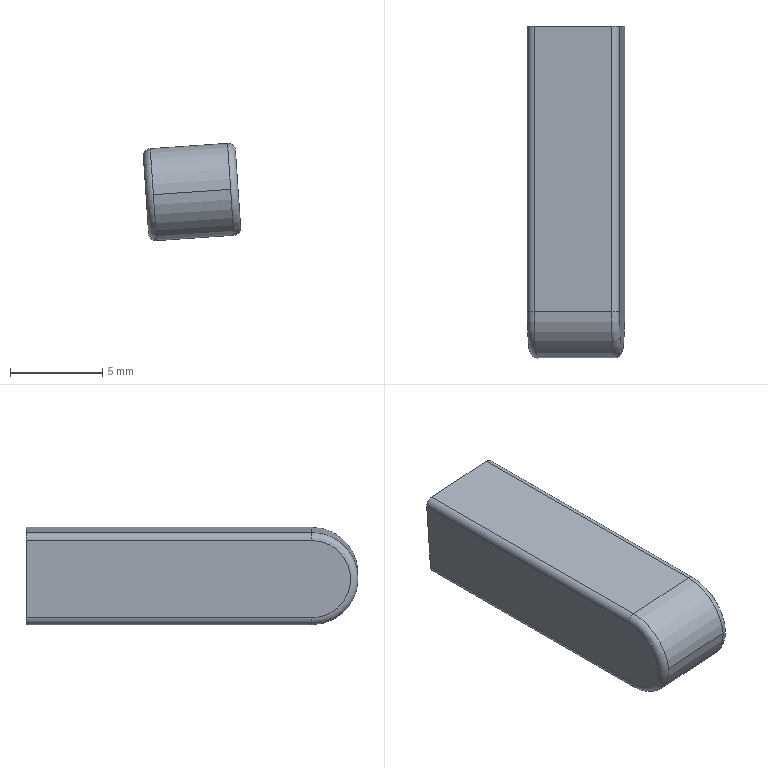Component | SolidWorks | GB_T1096-1979PlainParallelKeyC-type5_18-2 | 1 solid | 13 faces | box 5.28 x 18 x 5.28 mm | volume 434 mm3 | cylinder 6 | plane 5 | torus 2 | commonest cylinder face diameters 0.8 x4 5 x2
build123d program:
from build123d import *

# Parameters (mm, degrees)
BASE_EXTRUDE_DEPTH = 5
FILLET1_R          = 0.4


with BuildPart() as part:
    # Sketch1 → Base-Extrude (new body)
    with BuildSketch(Plane.XY):
        with BuildLine():
            Line((-9, 2.5), (6.5, 2.5))
            Line((6.5, 2.5), (6.5, -2.5))
            Line((6.5, -2.5), (-9, -2.5))
            ThreePointArc((-9, -2.5), (-11.5, 0), (-9, 2.5))
        make_face()
    extrude(amount=BASE_EXTRUDE_DEPTH)

    # Fillet1
    fillet1_edges = [part.edges().sort_by_distance(p)[0] for p in [
        (-11.5, 0, 5),
        (-1.25, -2.5, 5),
        (-1.25, -2.5, 0),
        (-11.5, 0, 0),
        (-1.25, 2.5, 0),
        (-1.25, 2.5, 5),
    ]]
    fillet(fillet1_edges, radius=FILLET1_R)


solid = part.part

# Placed as in the assembly
solid = solid.moved(Location((-24.351, 150.766, -166.303), (0, 86.093, 90)))
STEP:
#1=CARTESIAN_POINT('',(-0.7713,5.581,-6.633));
#2=VERTEX_POINT('',#1);
#3=CARTESIAN_POINT('',(-0.778,5.483,-6.535));
#4=VERTEX_POINT('',#3);
#5=CARTESIAN_POINT('',(-0.778,5.581,-6.535));
#6=DIRECTION('',(-0.9977,-0.,-0.06814));
#7=DIRECTION('',(0.,1.,0.));
#8=AXIS2_PLACEMENT_3D('',#5,#6,#7);
#9=CIRCLE('',#8,0.09843);
#10=EDGE_CURVE('',#2,#4,#9,.T.);
#11=ORIENTED_EDGE('',*,*,#10,.T.);
#12=CARTESIAN_POINT('',(-0.943,5.483,-6.546));
#13=VERTEX_POINT('',#12);
#14=CARTESIAN_POINT('',(-0.7623,5.483,-6.534));
#15=DIRECTION('',(-0.9977,-0.,-0.06814));
#16=VECTOR('',#15,39.37);
#17=LINE('',#14,#16);
#18=EDGE_CURVE('',#4,#13,#17,.T.);
#19=ORIENTED_EDGE('',*,*,#18,.T.);
#20=CARTESIAN_POINT('',(-0.9363,5.581,-6.644));
#21=VERTEX_POINT('',#20);
#22=CARTESIAN_POINT('',(-0.943,5.581,-6.546));
#23=DIRECTION('',(0.9977,0.,0.06814));
#24=DIRECTION('',(0.,1.,0.));
#25=AXIS2_PLACEMENT_3D('',#22,#23,#24);
#26=CIRCLE('',#25,0.09843);
#27=EDGE_CURVE('',#13,#21,#26,.T.);
#28=ORIENTED_EDGE('',*,*,#27,.T.);
#29=CARTESIAN_POINT('',(-0.7556,5.581,-6.632));
#30=DIRECTION('',(-0.9977,-0.,-0.06814));
#31=VECTOR('',#30,39.37);
#32=LINE('',#29,#31);
#33=EDGE_CURVE('',#2,#21,#32,.T.);
#34=ORIENTED_EDGE('',*,*,#33,.F.);
#35=EDGE_LOOP('',(#11,#19,#28,#34));
#36=FACE_OUTER_BOUND('',#35,.T.);
#37=CARTESIAN_POINT('',(-0.7623,5.581,-6.534));
#38=DIRECTION('',(-0.9977,-0.,-0.06814));
#39=DIRECTION('',(0.,-1.,0.));
#40=AXIS2_PLACEMENT_3D('',#37,#38,#39);
#41=CYLINDRICAL_SURFACE('',#40,0.09843);
#42=ADVANCED_FACE('',(#36),#41,.T.);
#43=CARTESIAN_POINT('',(-0.7567,6.192,-6.616));
#44=VERTEX_POINT('',#43);
#45=CARTESIAN_POINT('',(-0.768,6.192,-6.451));
#46=VERTEX_POINT('',#45);
#47=CARTESIAN_POINT('',(-0.769,6.192,-6.436));
#48=DIRECTION('',(-0.06814,0.,0.9977));
#49=VECTOR('',#48,39.37);
#50=LINE('',#47,#49);
#51=EDGE_CURVE('',#44,#46,#50,.T.);
#52=ORIENTED_EDGE('',*,*,#51,.F.);
#53=CARTESIAN_POINT('',(-0.7713,6.192,-6.633));
#54=VERTEX_POINT('',#53);
#55=CARTESIAN_POINT('',(-0.7724,6.192,-6.617));
#56=DIRECTION('',(0.,1.,-0.));
#57=DIRECTION('',(0.9977,0.,0.06814));
#58=AXIS2_PLACEMENT_3D('',#55,#56,#57);
#59=CIRCLE('',#58,0.01575);
#60=EDGE_CURVE('',#44,#54,#59,.T.);
#61=ORIENTED_EDGE('',*,*,#60,.T.);
#62=CARTESIAN_POINT('',(-0.9363,6.192,-6.644));
#63=VERTEX_POINT('',#62);
#64=CARTESIAN_POINT('',(-0.7556,6.192,-6.632));
#65=DIRECTION('',(-0.9977,-0.,-0.06814));
#66=VECTOR('',#65,39.37);
#67=LINE('',#64,#66);
#68=EDGE_CURVE('',#54,#63,#67,.T.);
#69=ORIENTED_EDGE('',*,*,#68,.T.);
#70=CARTESIAN_POINT('',(-0.9531,6.192,-6.63));
#71=VERTEX_POINT('',#70);
#72=CARTESIAN_POINT('',(-0.9374,6.192,-6.629));
#73=DIRECTION('',(0.,1.,-0.));
#74=DIRECTION('',(0.9977,0.,0.06814));
#75=AXIS2_PLACEMENT_3D('',#72,#73,#74);
#76=CIRCLE('',#75,0.01575);
#77=EDGE_CURVE('',#63,#71,#76,.T.);
#78=ORIENTED_EDGE('',*,*,#77,.T.);
#79=CARTESIAN_POINT('',(-0.9643,6.192,-6.465));
#80=VERTEX_POINT('',#79);
#81=CARTESIAN_POINT('',(-0.9654,6.192,-6.449));
#82=DIRECTION('',(-0.06814,0.,0.9977));
#83=VECTOR('',#82,39.37);
#84=LINE('',#81,#83);
#85=EDGE_CURVE('',#71,#80,#84,.T.);
#86=ORIENTED_EDGE('',*,*,#85,.T.);
#87=CARTESIAN_POINT('',(-0.9497,6.192,-6.448));
#88=VERTEX_POINT('',#87);
#89=CARTESIAN_POINT('',(-0.9486,6.192,-6.464));
#90=DIRECTION('',(0.,1.,-0.));
#91=DIRECTION('',(0.9977,0.,0.06814));
#92=AXIS2_PLACEMENT_3D('',#89,#90,#91);
#93=CIRCLE('',#92,0.01575);
#94=EDGE_CURVE('',#80,#88,#93,.T.);
#95=ORIENTED_EDGE('',*,*,#94,.T.);
#96=CARTESIAN_POINT('',(-0.7847,6.192,-6.437));
#97=VERTEX_POINT('',#96);
#98=CARTESIAN_POINT('',(-0.769,6.192,-6.436));
#99=DIRECTION('',(-0.9977,-0.,-0.06814));
#100=VECTOR('',#99,39.37);
#101=LINE('',#98,#100);
#102=EDGE_CURVE('',#97,#88,#101,.T.);
#103=ORIENTED_EDGE('',*,*,#102,.F.);
#104=CARTESIAN_POINT('',(-0.7837,6.192,-6.453));
#105=DIRECTION('',(0.,1.,-0.));
#106=DIRECTION('',(0.9977,0.,0.06814));
#107=AXIS2_PLACEMENT_3D('',#104,#105,#106);
#108=CIRCLE('',#107,0.01575);
#109=EDGE_CURVE('',#97,#46,#108,.T.);
#110=ORIENTED_EDGE('',*,*,#109,.T.);
#111=EDGE_LOOP('',(#52,#61,#69,#78,#86,#95,#103,#110));
#112=FACE_OUTER_BOUND('',#111,.T.);
#113=CARTESIAN_POINT('',(-0.769,6.192,-6.436));
#114=DIRECTION('',(-0.,-1.,0.));
#115=DIRECTION('',(0.9977,0.,0.06814));
#116=AXIS2_PLACEMENT_3D('',#113,#114,#115);
#117=PLANE('',#116);
#118=ADVANCED_FACE('',(#112),#117,.F.);
#119=CARTESIAN_POINT('',(-0.7847,5.581,-6.437));
#120=VERTEX_POINT('',#119);
#121=CARTESIAN_POINT('',(-0.9497,5.581,-6.448));
#122=VERTEX_POINT('',#121);
#123=CARTESIAN_POINT('',(-0.769,5.581,-6.436));
#124=DIRECTION('',(-0.9977,-0.,-0.06814));
#125=VECTOR('',#124,39.37);
#126=LINE('',#123,#125);
#127=EDGE_CURVE('',#120,#122,#126,.T.);
#128=ORIENTED_EDGE('',*,*,#127,.F.);
#129=CARTESIAN_POINT('',(-0.7847,6.192,-6.437));
#130=DIRECTION('',(0.,1.,-0.));
#131=VECTOR('',#130,39.37);
#132=LINE('',#129,#131);
#133=EDGE_CURVE('',#120,#97,#132,.T.);
#134=ORIENTED_EDGE('',*,*,#133,.T.);
#135=ORIENTED_EDGE('',*,*,#102,.T.);
#136=CARTESIAN_POINT('',(-0.9497,5.581,-6.448));
#137=DIRECTION('',(-0.,-1.,0.));
#138=VECTOR('',#137,39.37);
#139=LINE('',#136,#138);
#140=EDGE_CURVE('',#88,#122,#139,.T.);
#141=ORIENTED_EDGE('',*,*,#140,.T.);
#142=EDGE_LOOP('',(#128,#134,#135,#141));
#143=FACE_OUTER_BOUND('',#142,.T.);
#144=CARTESIAN_POINT('',(-0.769,5.581,-6.436));
#145=DIRECTION('',(0.06814,-0.,-0.9977));
#146=DIRECTION('',(-0.9977,-0.,-0.06814));
#147=AXIS2_PLACEMENT_3D('',#144,#145,#146);
#148=PLANE('',#147);
#149=ADVANCED_FACE('',(#143),#148,.F.);
#150=ORIENTED_EDGE('',*,*,#18,.F.);
#151=CARTESIAN_POINT('',(-0.778,5.581,-6.535));
#152=DIRECTION('',(-0.9977,-0.,-0.06814));
#153=DIRECTION('',(0.,1.,0.));
#154=AXIS2_PLACEMENT_3D('',#151,#152,#153);
#155=CIRCLE('',#154,0.09843);
#156=EDGE_CURVE('',#4,#120,#155,.T.);
#157=ORIENTED_EDGE('',*,*,#156,.T.);
#158=ORIENTED_EDGE('',*,*,#127,.T.);
#159=CARTESIAN_POINT('',(-0.943,5.581,-6.546));
#160=DIRECTION('',(0.9977,0.,0.06814));
#161=DIRECTION('',(0.,1.,0.));
#162=AXIS2_PLACEMENT_3D('',#159,#160,#161);
#163=CIRCLE('',#162,0.09843);
#164=EDGE_CURVE('',#122,#13,#163,.T.);
#165=ORIENTED_EDGE('',*,*,#164,.T.);
#166=EDGE_LOOP('',(#150,#157,#158,#165));
#167=FACE_OUTER_BOUND('',#166,.T.);
#168=CARTESIAN_POINT('',(-0.7623,5.581,-6.534));
#169=DIRECTION('',(-0.9977,-0.,-0.06814));
#170=DIRECTION('',(0.,-1.,0.));
#171=AXIS2_PLACEMENT_3D('',#168,#169,#170);
#172=CYLINDRICAL_SURFACE('',#171,0.09843);
#173=ADVANCED_FACE('',(#167),#172,.T.);
#174=ORIENTED_EDGE('',*,*,#68,.F.);
#175=CARTESIAN_POINT('',(-0.7713,5.581,-6.633));
#176=DIRECTION('',(-0.,-1.,0.));
#177=VECTOR('',#176,39.37);
#178=LINE('',#175,#177);
#179=EDGE_CURVE('',#54,#2,#178,.T.);
#180=ORIENTED_EDGE('',*,*,#179,.T.);
#181=ORIENTED_EDGE('',*,*,#33,.T.);
#182=CARTESIAN_POINT('',(-0.9363,5.581,-6.644));
#183=DIRECTION('',(0.,1.,-0.));
#184=VECTOR('',#183,39.37);
#185=LINE('',#182,#184);
#186=EDGE_CURVE('',#21,#63,#185,.T.);
#187=ORIENTED_EDGE('',*,*,#186,.T.);
#188=EDGE_LOOP('',(#174,#180,#181,#187));
#189=FACE_OUTER_BOUND('',#188,.T.);
#190=CARTESIAN_POINT('',(-0.7556,5.581,-6.632));
#191=DIRECTION('',(-0.06814,0.,0.9977));
#192=DIRECTION('',(0.9977,0.,0.06814));
#193=AXIS2_PLACEMENT_3D('',#190,#191,#192);
#194=PLANE('',#193);
#195=ADVANCED_FACE('',(#189),#194,.F.);
#196=CARTESIAN_POINT('',(-0.768,5.581,-6.451));
#197=VERTEX_POINT('',#196);
#198=CARTESIAN_POINT('',(-0.7567,5.581,-6.616));
#199=VERTEX_POINT('',#198);
#200=CARTESIAN_POINT('',(-0.7623,5.581,-6.534));
#201=DIRECTION('',(0.9977,0.,0.06814));
#202=DIRECTION('',(0.,1.,0.));
#203=AXIS2_PLACEMENT_3D('',#200,#201,#202);
#204=CIRCLE('',#203,0.08268);
#205=EDGE_CURVE('',#197,#199,#204,.T.);
#206=ORIENTED_EDGE('',*,*,#205,.T.);
#207=CARTESIAN_POINT('',(-0.7567,6.192,-6.616));
#208=DIRECTION('',(0.,1.,-0.));
#209=VECTOR('',#208,39.37);
#210=LINE('',#207,#209);
#211=EDGE_CURVE('',#199,#44,#210,.T.);
#212=ORIENTED_EDGE('',*,*,#211,.T.);
#213=ORIENTED_EDGE('',*,*,#51,.T.);
#214=CARTESIAN_POINT('',(-0.768,5.581,-6.451));
#215=DIRECTION('',(-0.,-1.,0.));
#216=VECTOR('',#215,39.37);
#217=LINE('',#214,#216);
#218=EDGE_CURVE('',#46,#197,#217,.T.);
#219=ORIENTED_EDGE('',*,*,#218,.T.);
#220=EDGE_LOOP('',(#206,#212,#213,#219));
#221=FACE_OUTER_BOUND('',#220,.T.);
#222=CARTESIAN_POINT('',(-0.7623,5.581,-6.534));
#223=DIRECTION('',(0.9977,0.,0.06814));
#224=DIRECTION('',(0.,1.,-0.));
#225=AXIS2_PLACEMENT_3D('',#222,#223,#224);
#226=PLANE('',#225);
#227=ADVANCED_FACE('',(#221),#226,.T.);
#228=CARTESIAN_POINT('',(-0.9531,5.581,-6.63));
#229=VERTEX_POINT('',#228);
#230=CARTESIAN_POINT('',(-0.9643,5.581,-6.465));
#231=VERTEX_POINT('',#230);
#232=CARTESIAN_POINT('',(-0.9587,5.581,-6.547));
#233=DIRECTION('',(-0.9977,-0.,-0.06814));
#234=DIRECTION('',(0.,1.,0.));
#235=AXIS2_PLACEMENT_3D('',#232,#233,#234);
#236=CIRCLE('',#235,0.08268);
#237=EDGE_CURVE('',#229,#231,#236,.T.);
#238=ORIENTED_EDGE('',*,*,#237,.T.);
#239=CARTESIAN_POINT('',(-0.9643,5.581,-6.465));
#240=DIRECTION('',(0.,1.,-0.));
#241=VECTOR('',#240,39.37);
#242=LINE('',#239,#241);
#243=EDGE_CURVE('',#231,#80,#242,.T.);
#244=ORIENTED_EDGE('',*,*,#243,.T.);
#245=ORIENTED_EDGE('',*,*,#85,.F.);
#246=CARTESIAN_POINT('',(-0.9531,5.581,-6.63));
#247=DIRECTION('',(-0.,-1.,0.));
#248=VECTOR('',#247,39.37);
#249=LINE('',#246,#248);
#250=EDGE_CURVE('',#71,#229,#249,.T.);
#251=ORIENTED_EDGE('',*,*,#250,.T.);
#252=EDGE_LOOP('',(#238,#244,#245,#251));
#253=FACE_OUTER_BOUND('',#252,.T.);
#254=CARTESIAN_POINT('',(-0.9587,5.581,-6.547));
#255=DIRECTION('',(0.9977,0.,0.06814));
#256=DIRECTION('',(0.,1.,-0.));
#257=AXIS2_PLACEMENT_3D('',#254,#255,#256);
#258=PLANE('',#257);
#259=ADVANCED_FACE('',(#253),#258,.F.);
#260=ORIENTED_EDGE('',*,*,#109,.F.);
#261=ORIENTED_EDGE('',*,*,#133,.F.);
#262=CARTESIAN_POINT('',(-0.7837,5.581,-6.453));
#263=DIRECTION('',(-0.,-1.,0.));
#264=DIRECTION('',(0.9977,0.,0.06814));
#265=AXIS2_PLACEMENT_3D('',#262,#263,#264);
#266=CIRCLE('',#265,0.01575);
#267=EDGE_CURVE('',#197,#120,#266,.T.);
#268=ORIENTED_EDGE('',*,*,#267,.F.);
#269=ORIENTED_EDGE('',*,*,#218,.F.);
#270=EDGE_LOOP('',(#260,#261,#268,#269));
#271=FACE_OUTER_BOUND('',#270,.T.);
#272=CARTESIAN_POINT('',(-0.7837,5.581,-6.453));
#273=DIRECTION('',(0.,1.,-0.));
#274=DIRECTION('',(-0.9977,0.,-0.06814));
#275=AXIS2_PLACEMENT_3D('',#272,#273,#274);
#276=CYLINDRICAL_SURFACE('',#275,0.01575);
#277=ADVANCED_FACE('',(#271),#276,.T.);
#278=ORIENTED_EDGE('',*,*,#267,.T.);
#279=ORIENTED_EDGE('',*,*,#156,.F.);
#280=ORIENTED_EDGE('',*,*,#10,.F.);
#281=CARTESIAN_POINT('',(-0.7724,5.581,-6.617));
#282=DIRECTION('',(0.,1.,-0.));
#283=DIRECTION('',(-0.9977,0.,-0.06814));
#284=AXIS2_PLACEMENT_3D('',#281,#282,#283);
#285=CIRCLE('',#284,0.01575);
#286=EDGE_CURVE('',#199,#2,#285,.T.);
#287=ORIENTED_EDGE('',*,*,#286,.F.);
#288=ORIENTED_EDGE('',*,*,#205,.F.);
#289=EDGE_LOOP('',(#278,#279,#280,#287,#288));
#290=FACE_OUTER_BOUND('',#289,.T.);
#291=CARTESIAN_POINT('',(-0.778,5.581,-6.535));
#292=DIRECTION('',(0.9977,0.,0.06814));
#293=DIRECTION('',(-0.,1.,-0.));
#294=AXIS2_PLACEMENT_3D('',#291,#292,#293);
#295=TOROIDAL_SURFACE('',#294,0.08268,0.01575);
#296=ADVANCED_FACE('',(#290),#295,.T.);
#297=ORIENTED_EDGE('',*,*,#286,.T.);
#298=ORIENTED_EDGE('',*,*,#179,.F.);
#299=ORIENTED_EDGE('',*,*,#60,.F.);
#300=ORIENTED_EDGE('',*,*,#211,.F.);
#301=EDGE_LOOP('',(#297,#298,#299,#300));
#302=FACE_OUTER_BOUND('',#301,.T.);
#303=CARTESIAN_POINT('',(-0.7724,5.581,-6.617));
#304=DIRECTION('',(-0.,-1.,0.));
#305=DIRECTION('',(0.9977,0.,0.06814));
#306=AXIS2_PLACEMENT_3D('',#303,#304,#305);
#307=CYLINDRICAL_SURFACE('',#306,0.01575);
#308=ADVANCED_FACE('',(#302),#307,.T.);
#309=ORIENTED_EDGE('',*,*,#77,.F.);
#310=ORIENTED_EDGE('',*,*,#186,.F.);
#311=CARTESIAN_POINT('',(-0.9374,5.581,-6.629));
#312=DIRECTION('',(-0.,-1.,0.));
#313=DIRECTION('',(0.9977,0.,0.06814));
#314=AXIS2_PLACEMENT_3D('',#311,#312,#313);
#315=CIRCLE('',#314,0.01575);
#316=EDGE_CURVE('',#229,#21,#315,.T.);
#317=ORIENTED_EDGE('',*,*,#316,.F.);
#318=ORIENTED_EDGE('',*,*,#250,.F.);
#319=EDGE_LOOP('',(#309,#310,#317,#318));
#320=FACE_OUTER_BOUND('',#319,.T.);
#321=CARTESIAN_POINT('',(-0.9374,5.581,-6.629));
#322=DIRECTION('',(0.,1.,-0.));
#323=DIRECTION('',(-0.9977,0.,-0.06814));
#324=AXIS2_PLACEMENT_3D('',#321,#322,#323);
#325=CYLINDRICAL_SURFACE('',#324,0.01575);
#326=ADVANCED_FACE('',(#320),#325,.T.);
#327=ORIENTED_EDGE('',*,*,#316,.T.);
#328=ORIENTED_EDGE('',*,*,#27,.F.);
#329=ORIENTED_EDGE('',*,*,#164,.F.);
#330=CARTESIAN_POINT('',(-0.9486,5.581,-6.464));
#331=DIRECTION('',(0.,1.,-0.));
#332=DIRECTION('',(-0.9977,0.,-0.06814));
#333=AXIS2_PLACEMENT_3D('',#330,#331,#332);
#334=CIRCLE('',#333,0.01575);
#335=EDGE_CURVE('',#231,#122,#334,.T.);
#336=ORIENTED_EDGE('',*,*,#335,.F.);
#337=ORIENTED_EDGE('',*,*,#237,.F.);
#338=EDGE_LOOP('',(#327,#328,#329,#336,#337));
#339=FACE_OUTER_BOUND('',#338,.T.);
#340=CARTESIAN_POINT('',(-0.943,5.581,-6.546));
#341=DIRECTION('',(0.9977,0.,0.06814));
#342=DIRECTION('',(-0.,1.,-0.));
#343=AXIS2_PLACEMENT_3D('',#340,#341,#342);
#344=TOROIDAL_SURFACE('',#343,0.08268,0.01575);
#345=ADVANCED_FACE('',(#339),#344,.T.);
#346=ORIENTED_EDGE('',*,*,#94,.F.);
#347=ORIENTED_EDGE('',*,*,#243,.F.);
#348=ORIENTED_EDGE('',*,*,#335,.T.);
#349=ORIENTED_EDGE('',*,*,#140,.F.);
#350=EDGE_LOOP('',(#346,#347,#348,#349));
#351=FACE_OUTER_BOUND('',#350,.T.);
#352=CARTESIAN_POINT('',(-0.9486,5.581,-6.464));
#353=DIRECTION('',(-0.,-1.,0.));
#354=DIRECTION('',(0.9977,0.,0.06814));
#355=AXIS2_PLACEMENT_3D('',#352,#353,#354);
#356=CYLINDRICAL_SURFACE('',#355,0.01575);
#357=ADVANCED_FACE('',(#351),#356,.T.);
#358=CLOSED_SHELL('',(#42,#118,#149,#173,#195,#227,#259,#277,#296,#308,#326,#345,#357));
#359=MANIFOLD_SOLID_BREP('',#358);
#360=CARTESIAN_POINT('',(0.,0.,0.));
#361=DIRECTION('',(0.,0.,1.));
#362=DIRECTION('',(1.,0.,0.));
#363=AXIS2_PLACEMENT_3D('',#360,#361,#362);
#364=(LENGTH_UNIT()NAMED_UNIT(*)SI_UNIT($,.METRE.));
#365=LENGTH_MEASURE_WITH_UNIT(LENGTH_MEASURE(0.0254),#364);
#366=DIMENSIONAL_EXPONENTS(1.,0.,0.,0.,0.,0.,0.);
#367=(CONVERSION_BASED_UNIT('',#365)LENGTH_UNIT()NAMED_UNIT(#366));
#368=UNCERTAINTY_MEASURE_WITH_UNIT(LENGTH_MEASURE(0.00001),#367,'','');
#369=(NAMED_UNIT(*)PLANE_ANGLE_UNIT()SI_UNIT($,.RADIAN.));
#370=(NAMED_UNIT(*)SI_UNIT($,.STERADIAN.)SOLID_ANGLE_UNIT());
#371=(GEOMETRIC_REPRESENTATION_CONTEXT(3)GLOBAL_UNCERTAINTY_ASSIGNED_CONTEXT((#368))GLOBAL_UNIT_ASSIGNED_CONTEXT((#367,#369,#370))REPRESENTATION_CONTEXT('',''));
#372=ADVANCED_BREP_SHAPE_REPRESENTATION('',(#359,#363),#371);
#373=COLOUR_RGB('',0.7922,0.8196,0.9333);
#374=FILL_AREA_STYLE_COLOUR('',#373);
#375=FILL_AREA_STYLE('',(#374));
#376=SURFACE_STYLE_FILL_AREA(#375);
#377=SURFACE_SIDE_STYLE('',(#376));
#378=SURFACE_STYLE_USAGE(.BOTH.,#377);
#379=PRESENTATION_STYLE_ASSIGNMENT((#378));
#380=STYLED_ITEM('',(#379),#359);
#381=PRESENTATION_LAYER_ASSIGNMENT('','',(#380));
#382=(LENGTH_UNIT()NAMED_UNIT(*)SI_UNIT($,.METRE.));
#383=LENGTH_MEASURE_WITH_UNIT(LENGTH_MEASURE(0.0254),#382);
#384=DIMENSIONAL_EXPONENTS(1.,0.,0.,0.,0.,0.,0.);
#385=(CONVERSION_BASED_UNIT('',#383)LENGTH_UNIT()NAMED_UNIT(#384));
#386=UNCERTAINTY_MEASURE_WITH_UNIT(LENGTH_MEASURE(0.00001),#385,'','');
#387=(NAMED_UNIT(*)PLANE_ANGLE_UNIT()SI_UNIT($,.RADIAN.));
#388=(NAMED_UNIT(*)SI_UNIT($,.STERADIAN.)SOLID_ANGLE_UNIT());
#389=(GEOMETRIC_REPRESENTATION_CONTEXT(3)GLOBAL_UNCERTAINTY_ASSIGNED_CONTEXT((#386))GLOBAL_UNIT_ASSIGNED_CONTEXT((#385,#387,#388))REPRESENTATION_CONTEXT('',''));
#390=MECHANICAL_DESIGN_GEOMETRIC_PRESENTATION_REPRESENTATION('',(#380),#389);